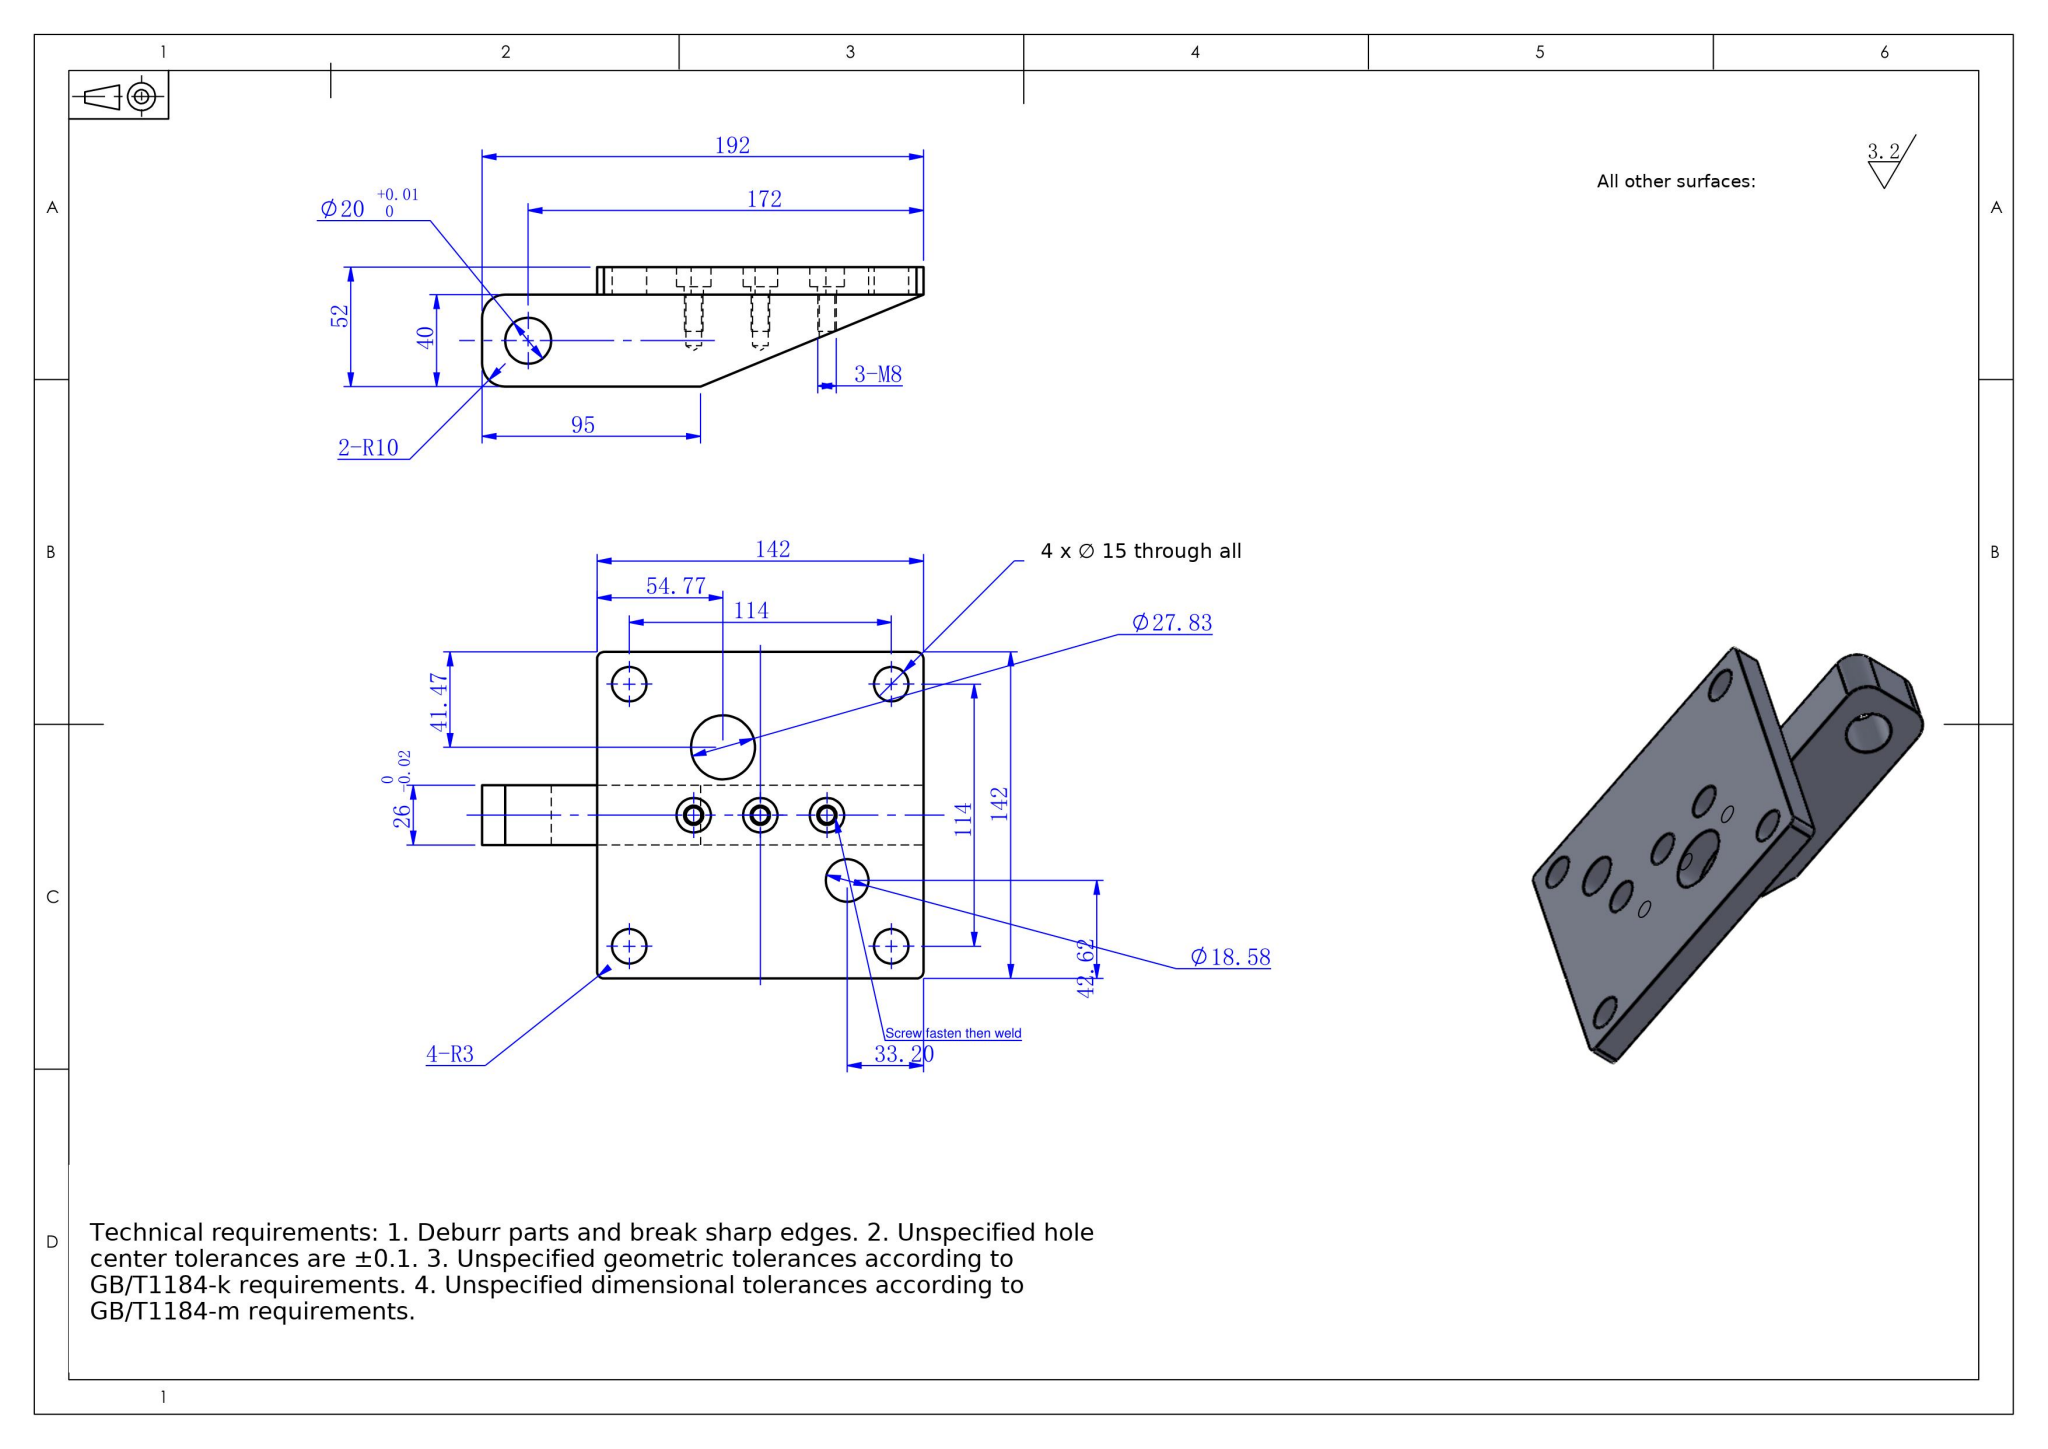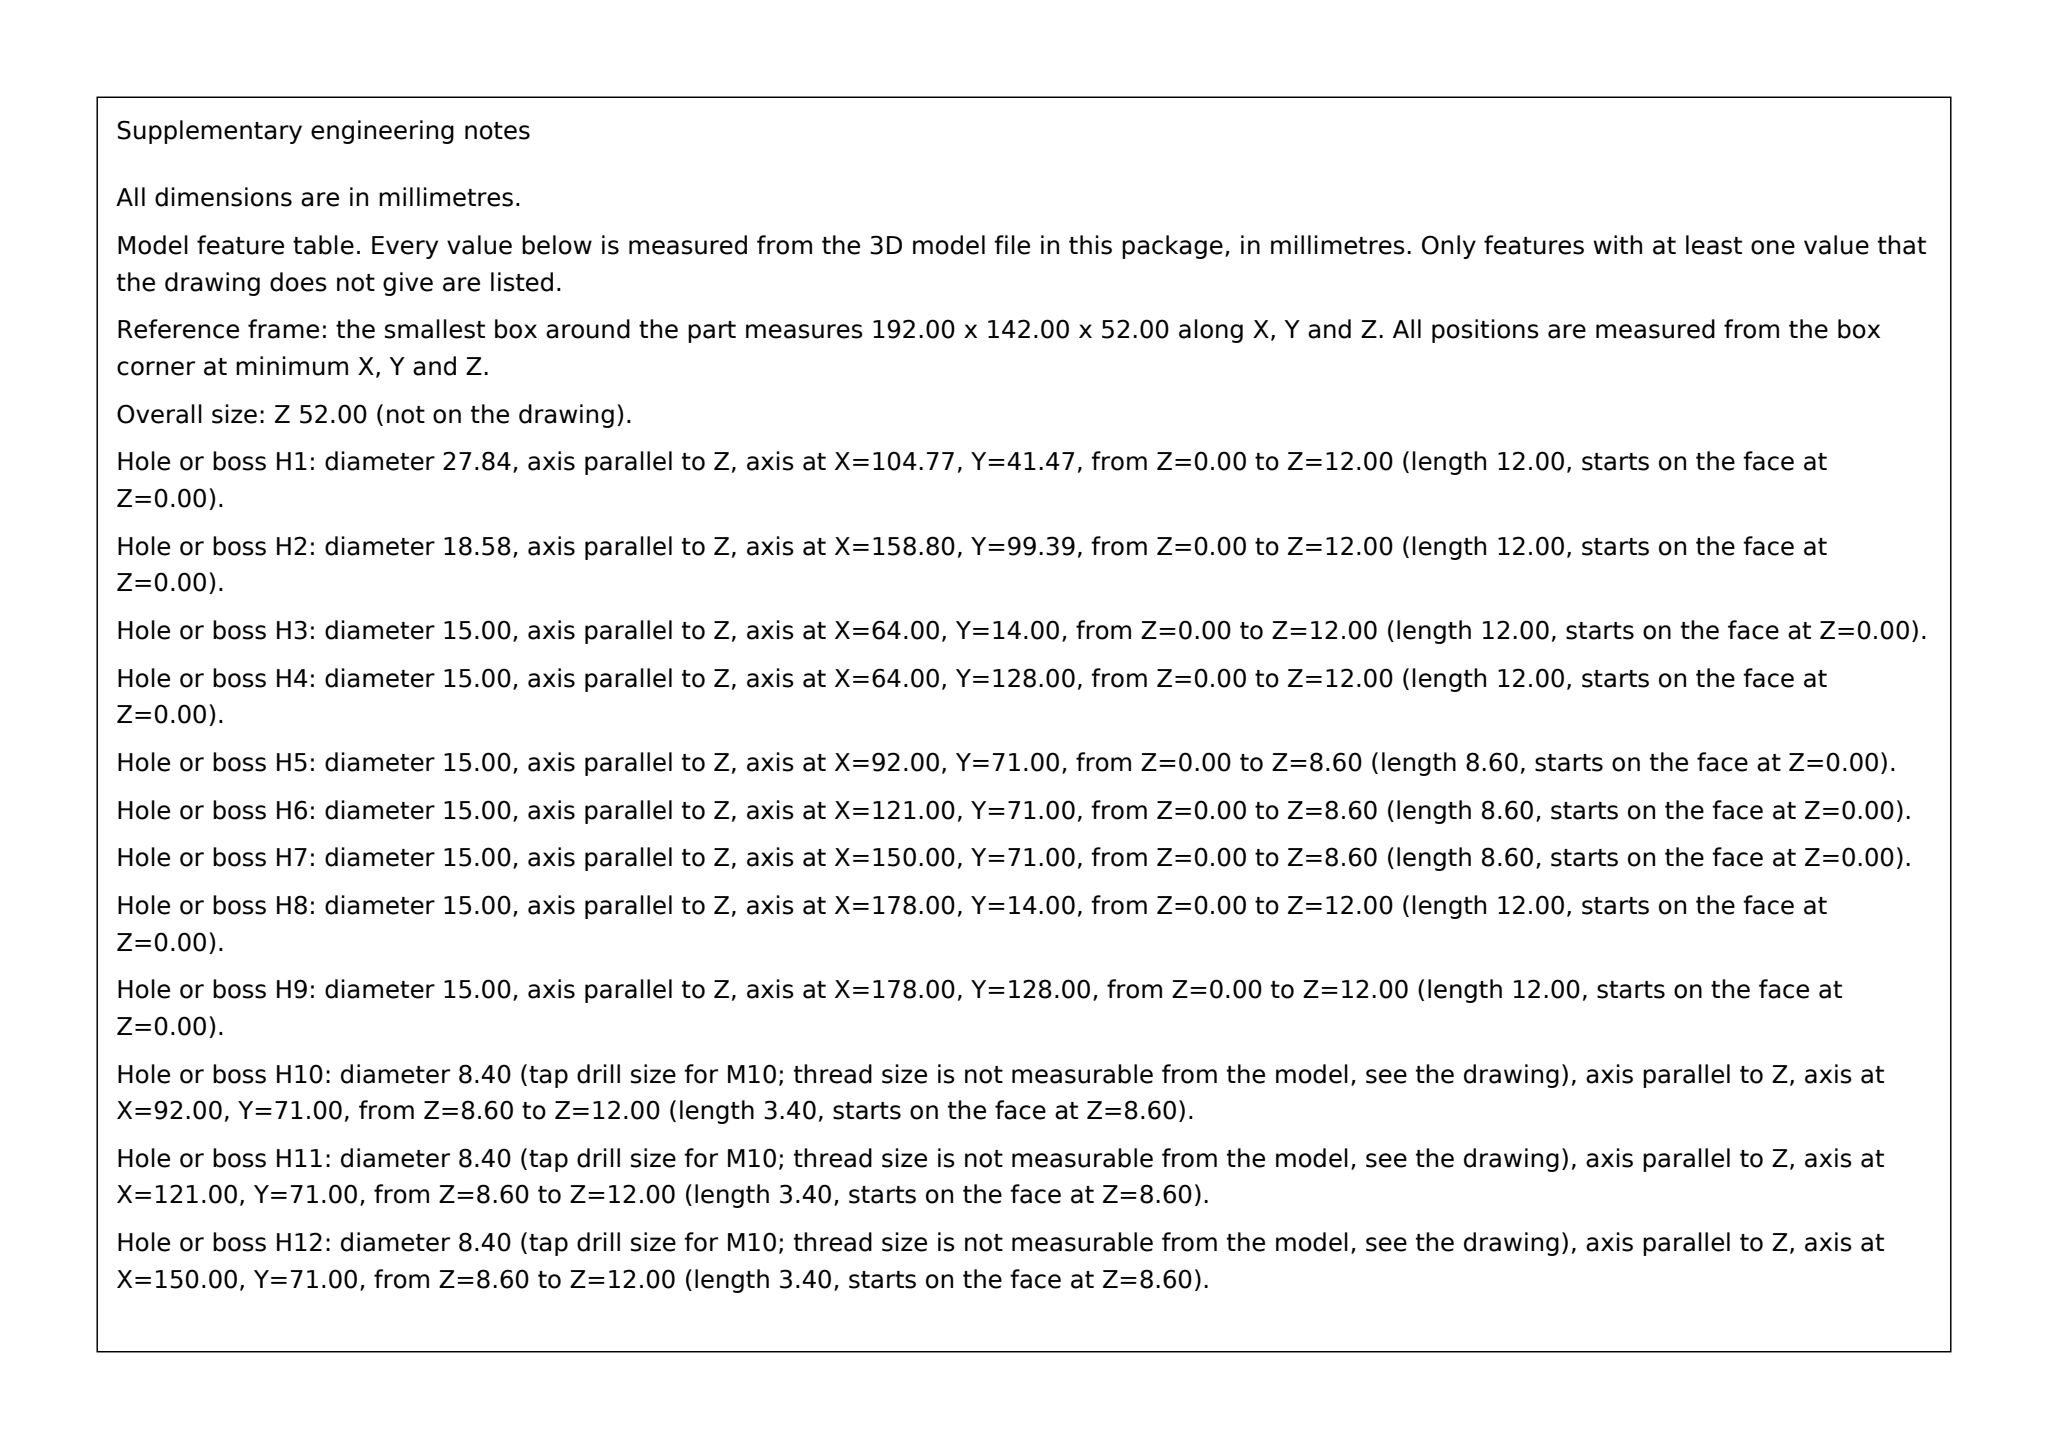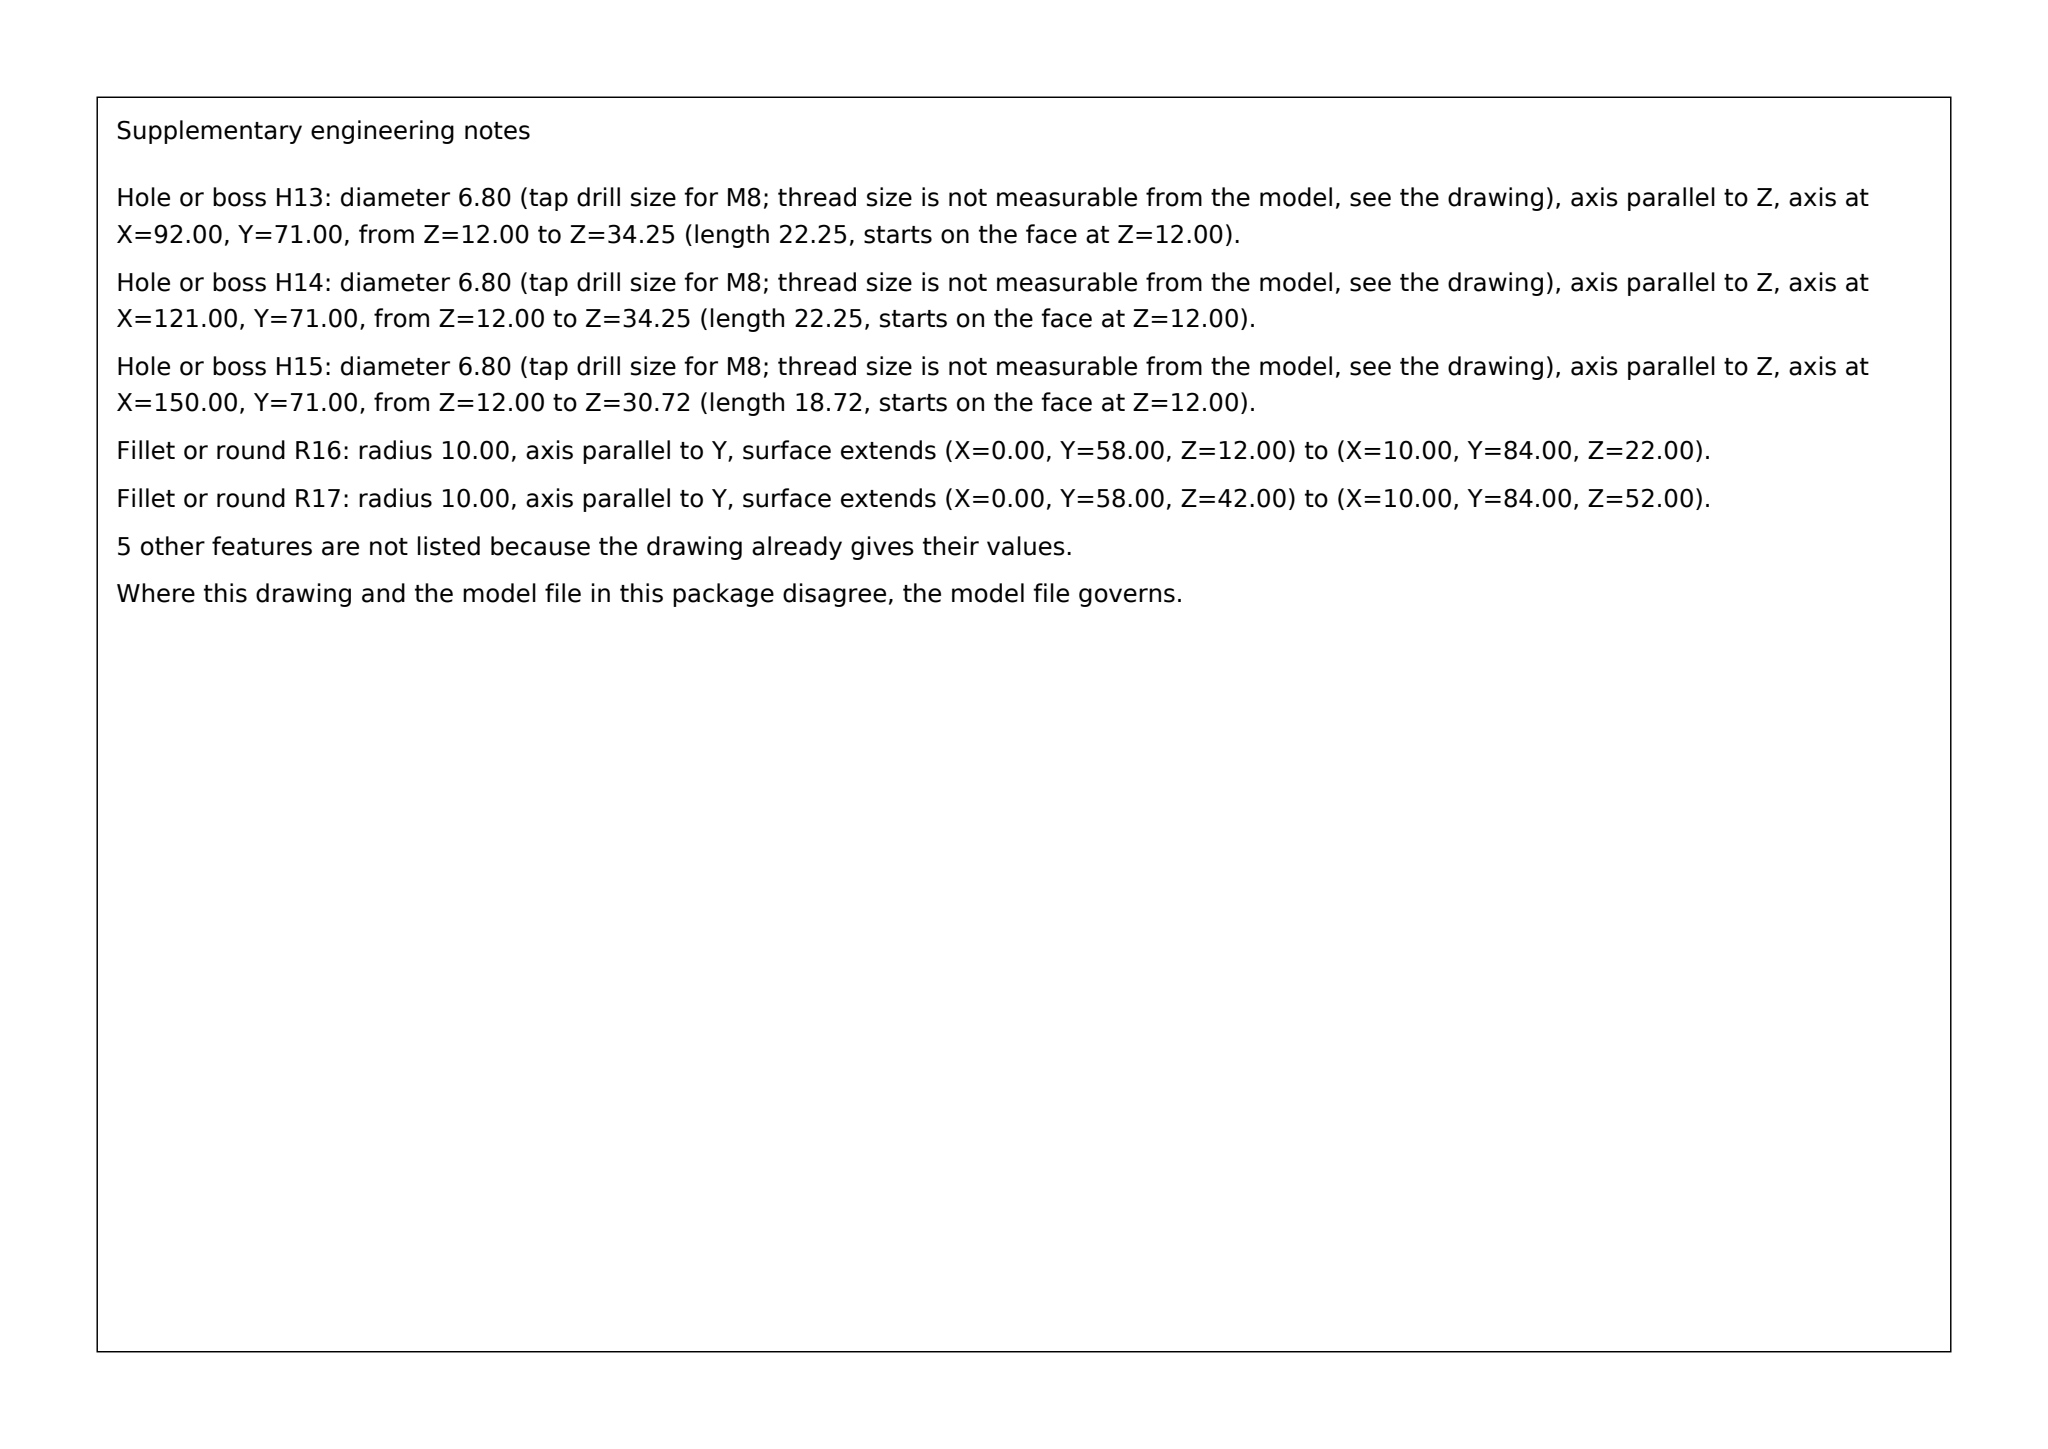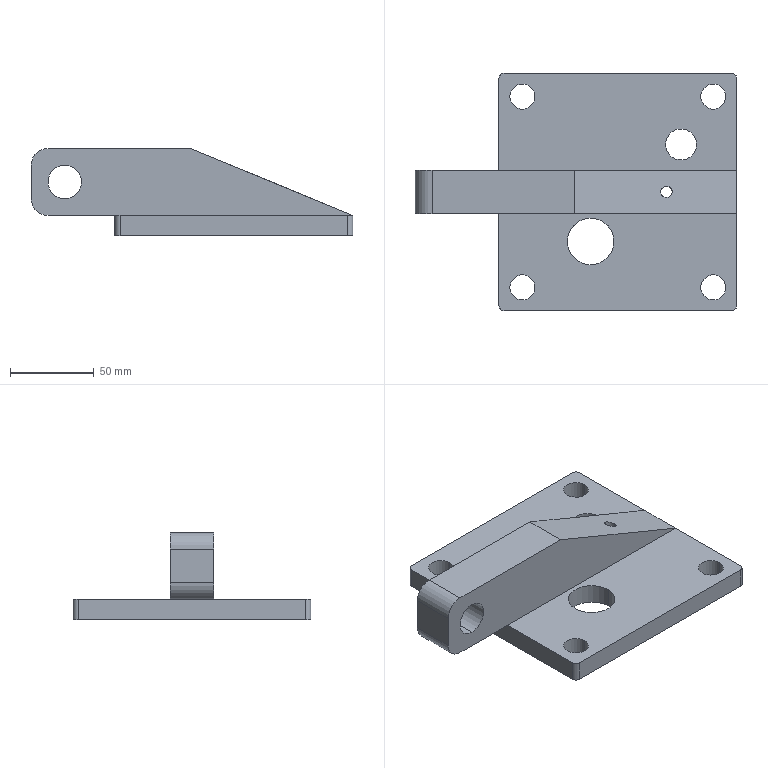Part | SolidWorks | mm | 1 solid | 61 faces | box 192 x 142 x 52 mm | volume 355375 mm3 | cylinder 38 | plane 19 | cone 4 | commonest cylinder face diameters 15 x14 6.8 x6 8.4 x6 20 x4 6 x4 18.584 x2 27.831 x2
build123d program:
from build123d import *

# Parameters (mm, degrees)
SKETCH1_W                                       = 142
SKETCH1_H                                       = 142
BOSS_EXTRUDE1_DEPTH                             = 12
SKETCH2_W                                       = 45
SKETCH2_H                                       = 26
BOSS_EXTRUDE2_DEPTH                             = 40
SKETCH3_W                                       = 40
SKETCH3_H                                       = 26
BOSS_EXTRUDE3_DEPTH                             = 50
FILLET3_R                                       = 10
BOSS_EXTRUDE4_DEPTH                             = 26
SKETCH5_R                                       = 10
CUT_EXTRUDE1_DEPTH                              = 171.487
F_10_5_10_5_DIAMETER_HOLE1_D                    = 15
FILLET4_R                                       = 3
M8_HEX_SOCKET_HEAD_CAP_SCREW_CBORE1_D           = 8.4
M8_HEX_SOCKET_HEAD_CAP_SCREW_CBORE1_DEPTH       = 11.999
M8_HEX_SOCKET_HEAD_CAP_SCREW_CBORE1_CBORE_D     = 15
M8_HEX_SOCKET_HEAD_CAP_SCREW_CBORE1_CBORE_DEPTH = 8.6
M8_TAPPED_HOLE1_D                               = 6.8
M8_TAPPED_HOLE1_DEPTH                           = 22.25
M8_TAPPED_HOLE1_TIP                             = 2.043
SKETCH13_R                                      = 9.292
SKETCH13_R_2                                    = 13.916
CUT_EXTRUDE2_DEPTH                              = 73


with BuildPart() as part:
    # Sketch1 → Boss-Extrude1 (new body)
    with BuildSketch(Plane.XY):
        with Locations((-17.946, -15.786)):
            Rectangle(SKETCH1_W, SKETCH1_H)
    extrude(amount=BOSS_EXTRUDE1_DEPTH)

    # Sketch2 → Boss-Extrude2 (add)
    with BuildSketch(Plane.XY.offset(12)):
        with Locations((-66.446, -15.786)):
            Rectangle(SKETCH2_W, SKETCH2_H)
    extrude(amount=BOSS_EXTRUDE2_DEPTH)

    # Sketch3 → Boss-Extrude3 (add)
    with BuildSketch(Plane.ZY.offset(88.946)):
        with Locations((32, -15.786)):
            Rectangle(SKETCH3_W, SKETCH3_H)
    extrude(amount=BOSS_EXTRUDE3_DEPTH)

    # Fillet3
    fillet3_edges = [part.edges().sort_by_distance(p)[0] for p in [
        (-138.946, -15.786, 52),
        (-138.946, -15.786, 12),
    ]]
    fillet(fillet3_edges, radius=FILLET3_R)

    # Sketch4 → Boss-Extrude4 (add)
    with BuildSketch(Plane(origin=(0, -2.786, 0), x_dir=(1, 0, 0), z_dir=(0, 1, 0))):
        Polygon((-43.946, -52), (53.054, -12), (-43.946, -12), align=None)
    extrude(amount=-BOSS_EXTRUDE4_DEPTH)

    # Sketch5 → Cut-Extrude1 (cut, through all)
    with BuildSketch(Plane(origin=(0, -2.786, 0), x_dir=(1, 0, 0), z_dir=(0, 1, 0))):
        with Locations(Location((-118.946, -32, 0), (0, 0, 270))):
            Circle(SKETCH5_R)
    extrude(amount=-CUT_EXTRUDE1_DEPTH, mode=Mode.SUBTRACT)

    # 10.5 _10.5_ Diameter Hole1 (through all)
    with Locations(Plane.XY.offset(12)):
        with Locations((-74.946, 41.214), (39.054, 41.214), (39.054, -72.786), (-74.946, -72.786)):
            Hole(F_10_5_10_5_DIAMETER_HOLE1_D / 2)

    # Fillet4
    fillet4_edges = [part.edges().sort_by_distance(p)[0] for p in [
        (53.054, 55.214, 6),
        (53.054, -86.786, 6),
        (-88.946, -86.786, 6),
        (-88.946, 55.214, 6),
    ]]
    fillet(fillet4_edges, radius=FILLET4_R)

    # M8 Hex Socket Head Cap Screw CBORE1
    with Locations(Plane(origin=(0, 0, 0), x_dir=(-1, 0, 0), z_dir=(0, 0, -1))):
        with Locations((46.946, -15.786), (-11.054, -15.786), (17.946, -15.786)):
            CounterBoreHole(M8_HEX_SOCKET_HEAD_CAP_SCREW_CBORE1_D / 2, M8_HEX_SOCKET_HEAD_CAP_SCREW_CBORE1_CBORE_D / 2, M8_HEX_SOCKET_HEAD_CAP_SCREW_CBORE1_CBORE_DEPTH, depth=M8_HEX_SOCKET_HEAD_CAP_SCREW_CBORE1_DEPTH)

    # M8 Tapped Hole1
    with Locations(Plane(origin=(0, 0, 12), x_dir=(-1, 0, 0), z_dir=(0, 0, -1))):
        with Locations((-11.054, -15.786), (17.946, -15.786), (46.946, -15.786)):
            Hole(M8_TAPPED_HOLE1_D / 2, depth=M8_TAPPED_HOLE1_DEPTH)
            with Locations((0, 0, -(M8_TAPPED_HOLE1_DEPTH + M8_TAPPED_HOLE1_TIP / 2))):  # 118° drill point
                Cone(0, M8_TAPPED_HOLE1_D / 2, M8_TAPPED_HOLE1_TIP, mode=Mode.SUBTRACT)

    # Sketch13 → Cut-Extrude2 (cut)
    with BuildSketch(Plane(origin=(0, 0, 0), x_dir=(-1, 0, 0), z_dir=(0, 0, -1))):
        with Locations((-19.853, 12.595)):
            Circle(SKETCH13_R)
        with Locations((34.18, -45.317)):
            Circle(SKETCH13_R_2)
    extrude(amount=-CUT_EXTRUDE2_DEPTH, mode=Mode.SUBTRACT)


solid = part.part